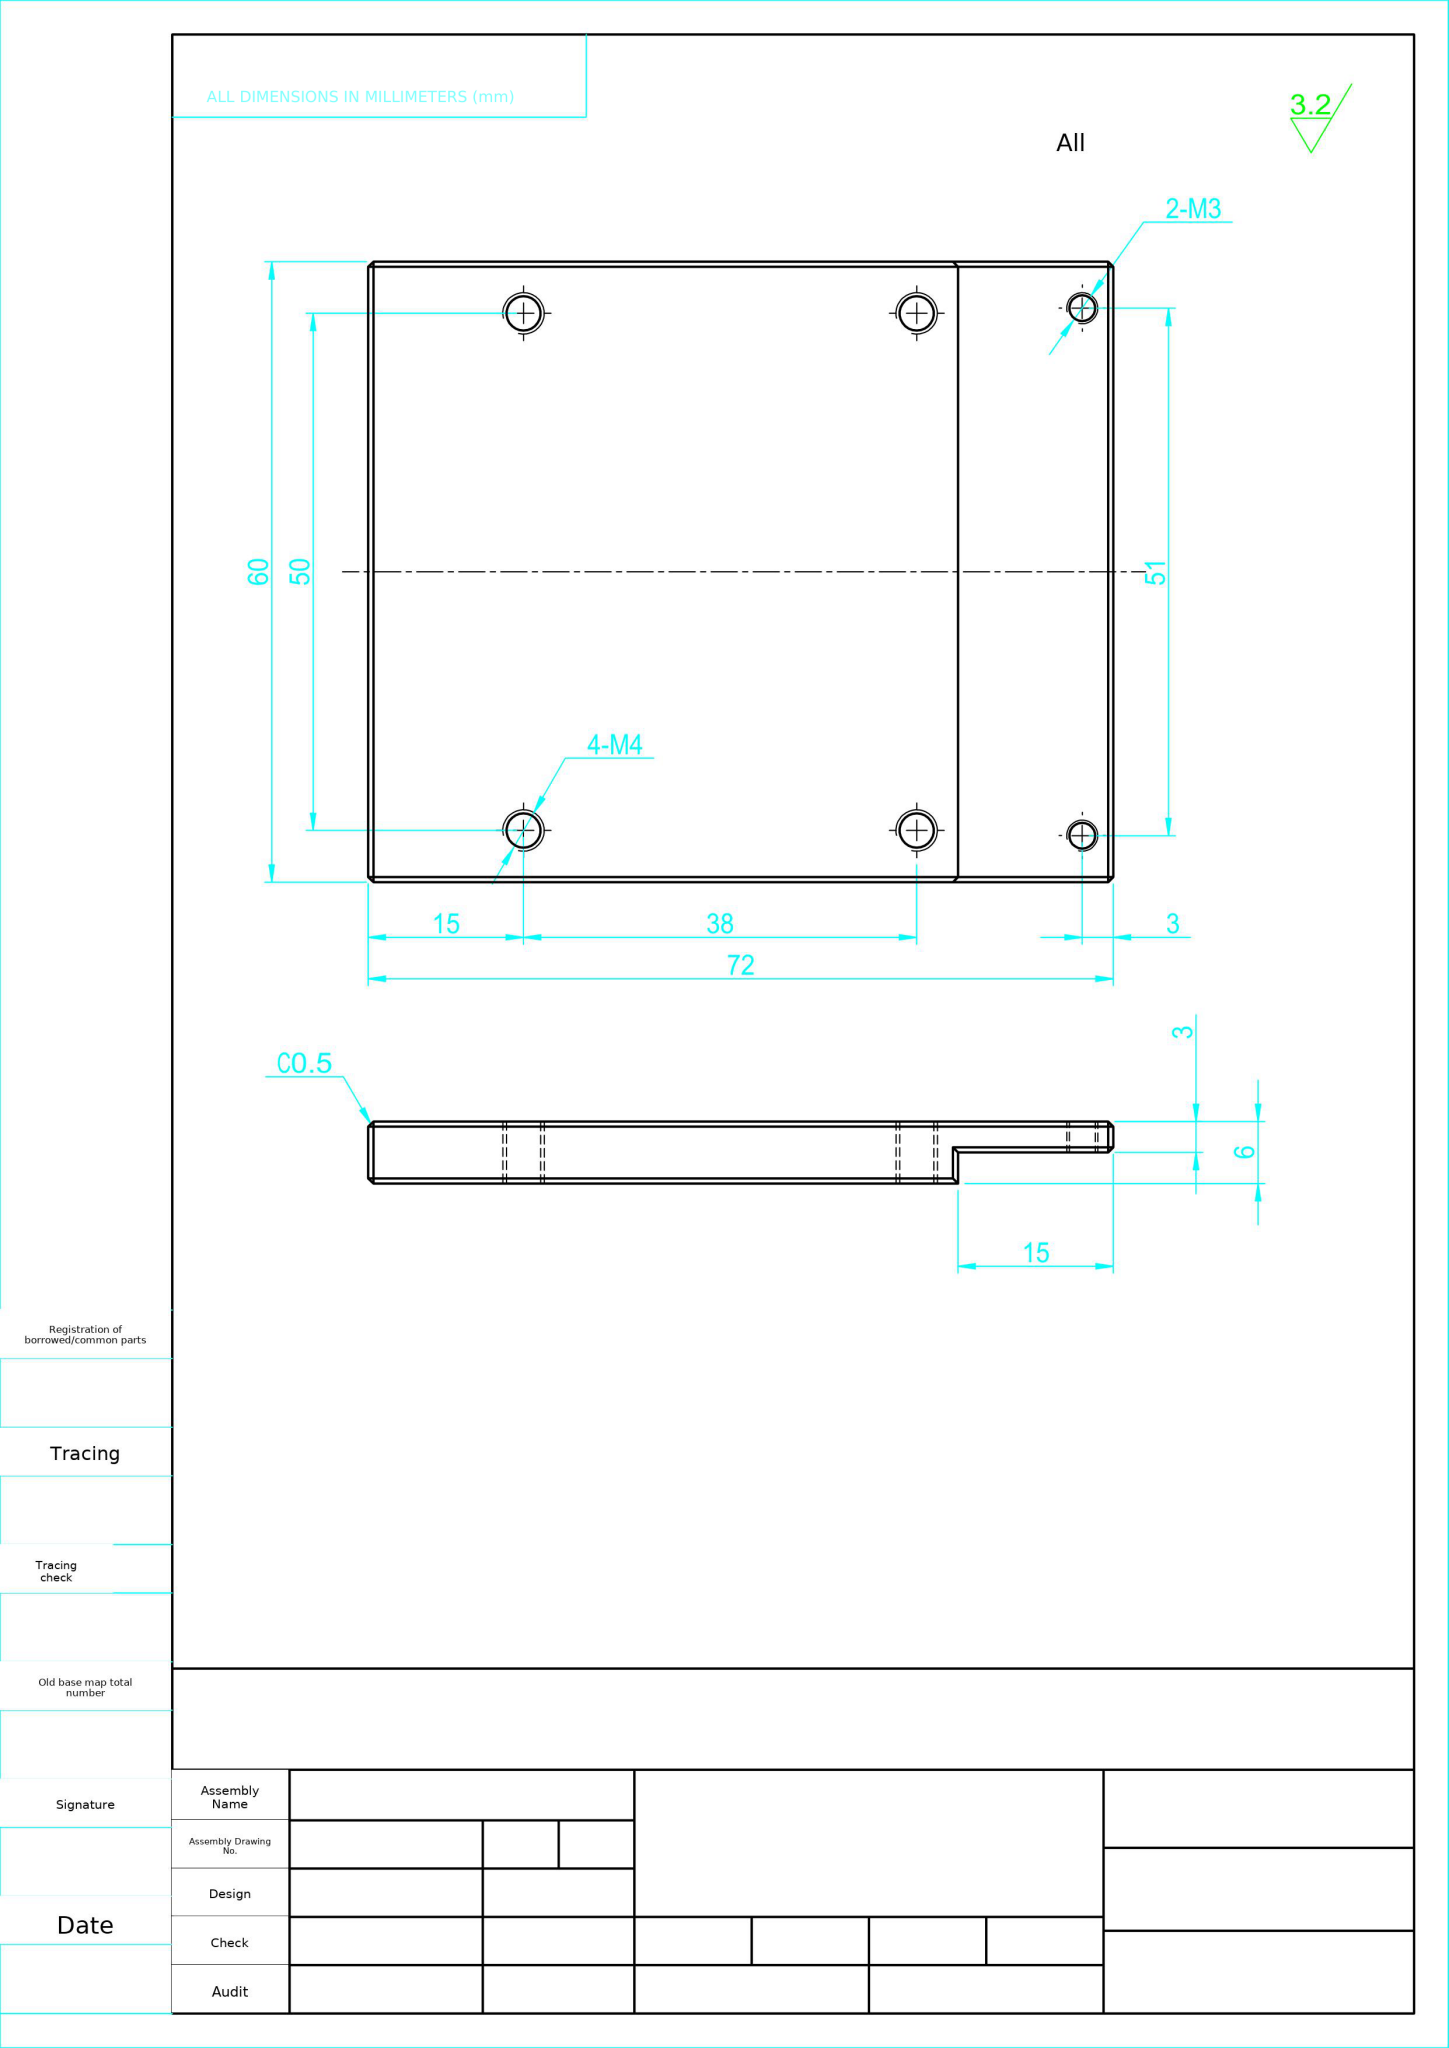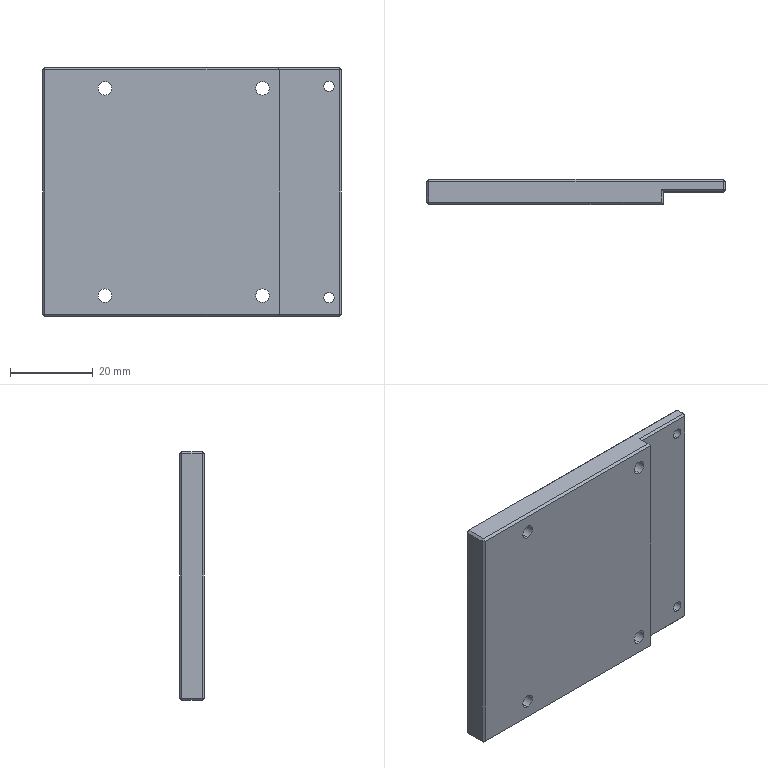Part | NX | mm | 1 solid | 44 faces | box 72 x 6 x 60 mm | volume 22917 mm3 | plane 32 | cylinder 12 | commonest cylinder face diameters 3.3 x8 2.5 x4